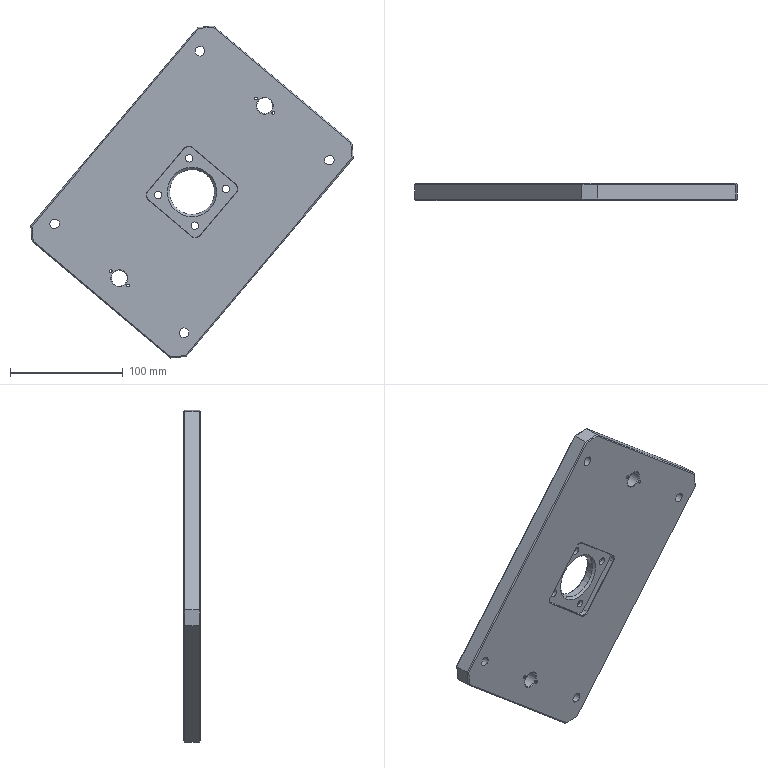Component | SolidWorks | 01GripperConnectionPlate-1 | 1 solid | 107 faces | box 285.83 x 15 x 294.29 mm | volume 624686 mm3 | cylinder 46 | plane 41 | cone 20 | commonest cylinder face diameters 2.5 x8 11 x8 6.6 x8 8.5 x8 14 x4 27 x4 10 x4 40 x2 | material Aviation Aluminum-7075
build123d program:
from build123d import *

# Parameters (mm, degrees)
SKETCH1_W                                          = 250
SKETCH1_H                                          = 180
BOSS_EXTRUDE1_DEPTH                                = 15
M10_TAPPED_HOLE1_D                                 = 8.5
SKETCH3_W                                          = 60
SKETCH3_H                                          = 60
CUT_EXTRUDE1_DEPTH                                 = 5
CHAMFER1_SIZE                                      = 10
FILLET1_R                                          = 5
CUT_EXTRUDE2_REACH                                 = 156.353
SKETCH4_R                                          = 20
CUT_EXTRUDE3_REACH                                 = 156.758
SKETCH5_R                                          = 5
HOLE_SIZE_ACCORDING_TO_TYPE_1_OF_HEXAG_D           = 6.6
HOLE_SIZE_ACCORDING_TO_TYPE_1_OF_HEXAG_CBORE_D     = 11
HOLE_SIZE_ACCORDING_TO_TYPE_1_OF_HEXAG_CBORE_DEPTH = 6.8
CIRPATTERN1_COUNT                                  = 4
CHAMFER2_SIZE                                      = 0.5
SKETCH7_R                                          = 13.5
CUT_EXTRUDE4_DEPTH                                 = 5
CUT_EXTRUDE5_REACH                                 = 156.353
SKETCH8_R                                          = 7
CHAMFER3_SIZE                                      = 0.5
M3_TAPPED_HOLE1_D                                  = 2.5
LPATTERN1_COUNT                                    = 2
LPATTERN1_PITCH                                    = 200
CHAMFER4_SIZE                                      = 1
CHAMFER5_SIZE                                      = 2


with BuildPart() as part:
    # Sketch1 → Boss-Extrude1 (new body)
    with BuildSketch(Plane.XY):
        Rectangle(SKETCH1_W, SKETCH1_H)
    extrude(amount=BOSS_EXTRUDE1_DEPTH)

    # M10 Tapped Hole1 (through all)
    with Locations(Plane(origin=(-100, 75, 15), x_dir=(1, 0, 0), z_dir=(0, 0, 1))):
        with Locations((0, 0), (0, -150), (200, -150), (200, 0)):
            Hole(M10_TAPPED_HOLE1_D / 2)

    # Sketch3 → Cut-Extrude1 (cut)
    with BuildSketch(Plane.XY.offset(15)):
        Rectangle(SKETCH3_W, SKETCH3_H)
    extrude(amount=-CUT_EXTRUDE1_DEPTH, mode=Mode.SUBTRACT)

    # Chamfer1
    chamfer1_edges = [part.edges().sort_by_distance(p)[0] for p in [
        (-125, 90, 7.5),
        (125, 90, 7.5),
        (125, -90, 7.5),
        (-125, -90, 7.5),
    ]]
    chamfer(chamfer1_edges, length=CHAMFER1_SIZE)

    # Fillet1
    fillet1_edges = [part.edges().sort_by_distance(p)[0] for p in [
        (-30, -30, 12.5),
        (-30, 30, 12.5),
        (30, 30, 12.5),
        (30, -30, 12.5),
    ]]
    fillet(fillet1_edges, radius=FILLET1_R)

    # Sketch4 → Cut-Extrude2 (cut, up to next)
    with BuildSketch(Plane.XY.offset(10), mode=Mode.PRIVATE) as cut_extrude2_sk1:
        Circle(SKETCH4_R)
    cut_extrude2_tool1 = extrude(cut_extrude2_sk1.sketch, amount=-CUT_EXTRUDE2_REACH, mode=Mode.PRIVATE) & part.part
    add(cut_extrude2_tool1.solids().sort_by_distance((0, 0, 10))[0], mode=Mode.SUBTRACT)

    # Sketch5 → Cut-Extrude3 (cut, up to next)
    with BuildSketch(Plane.XY.offset(15), mode=Mode.PRIVATE) as cut_extrude3_sk1:
        with Locations((-100, 0)):
            Circle(SKETCH5_R)
    cut_extrude3_tool1 = extrude(cut_extrude3_sk1.sketch, amount=-CUT_EXTRUDE3_REACH, mode=Mode.PRIVATE) & part.part
    # Sketch5 → Cut-Extrude3 (cut, up to next)
    with BuildSketch(Plane.XY.offset(15), mode=Mode.PRIVATE) as cut_extrude3_sk2:
        with Locations((100, 0)):
            Circle(SKETCH5_R)
    cut_extrude3_tool2 = extrude(cut_extrude3_sk2.sketch, amount=-CUT_EXTRUDE3_REACH, mode=Mode.PRIVATE) & part.part
    add(cut_extrude3_tool1.solids().sort_by_distance((-100, 0, 15))[0], mode=Mode.SUBTRACT)
    add(cut_extrude3_tool2.solids().sort_by_distance((100, 0, 15))[0], mode=Mode.SUBTRACT)

    # Hole Size _According to_ Type 1 of Hexag (through all)
    with Locations(Plane(origin=(21.213, 21.213, 0), x_dir=(-1, 0, 0), z_dir=(0, 0, -1))):
        with Locations((0, 0)):
            hole_size_according_to_type_1_of_hexag = CounterBoreHole(HOLE_SIZE_ACCORDING_TO_TYPE_1_OF_HEXAG_D / 2, HOLE_SIZE_ACCORDING_TO_TYPE_1_OF_HEXAG_CBORE_D / 2, HOLE_SIZE_ACCORDING_TO_TYPE_1_OF_HEXAG_CBORE_DEPTH)

    # CirPattern1: Hole Size _According to_ Type 1 of Hexag ×4 about axis
    cirpattern1_axis = Axis((0, 0, 0), (0, 0, 1))
    for i in range(1, CIRPATTERN1_COUNT):
        add(hole_size_according_to_type_1_of_hexag.rotate(cirpattern1_axis, i * 360 / CIRPATTERN1_COUNT), mode=Mode.SUBTRACT)

    # Chamfer2
    chamfer2_edges = [part.edges().sort_by_distance(p)[0] for p in [
        (30, 0, 15),
        (0, -30, 15),
        (-30, 0, 15),
        (0, 30, 15),
        (28.536, -28.536, 15),
        (-28.536, -28.536, 15),
        (-28.536, 28.536, 15),
        (28.536, 28.536, 15),
    ]]
    chamfer(chamfer2_edges, length=CHAMFER2_SIZE)

    # Sketch7 → Cut-Extrude4 (cut)
    with BuildSketch(Plane(origin=(0, 0, 0), x_dir=(-1, 0, 0), z_dir=(0, 0, -1))):
        with Locations((-100, 0)):
            Circle(SKETCH7_R)
        with Locations((100, 0)):
            Circle(SKETCH7_R)
    extrude(amount=-CUT_EXTRUDE4_DEPTH, mode=Mode.SUBTRACT)

    # Sketch8 → Cut-Extrude5 (cut, up to next)
    with BuildSketch(Plane(origin=(0, 0, 5), x_dir=(-1, 0, 0), z_dir=(0, 0, -1)), mode=Mode.PRIVATE) as cut_extrude5_sk1:
        with Locations((-100, 0)):
            Circle(SKETCH8_R)
    cut_extrude5_tool1 = extrude(cut_extrude5_sk1.sketch, amount=-CUT_EXTRUDE5_REACH, mode=Mode.PRIVATE) & part.part
    # Sketch8 → Cut-Extrude5 (cut, up to next)
    with BuildSketch(Plane(origin=(0, 0, 5), x_dir=(-1, 0, 0), z_dir=(0, 0, -1)), mode=Mode.PRIVATE) as cut_extrude5_sk2:
        with Locations((100, 0)):
            Circle(SKETCH8_R)
    cut_extrude5_tool2 = extrude(cut_extrude5_sk2.sketch, amount=-CUT_EXTRUDE5_REACH, mode=Mode.PRIVATE) & part.part
    add(cut_extrude5_tool1.solids().sort_by_distance((100, 0, 5))[0], mode=Mode.SUBTRACT)
    add(cut_extrude5_tool2.solids().sort_by_distance((-100, 0, 5))[0], mode=Mode.SUBTRACT)

    # Chamfer3
    chamfer3_edges = [part.edges().sort_by_distance(p)[0] for p in [
        (113.5, 0, 0),
        (-86.5, 0, 0),
        (107, 0, 15),
        (107, 0, 5),
        (-93, 0, 15),
        (-93, 0, 5),
    ]]
    chamfer(chamfer3_edges, length=CHAMFER3_SIZE)

    # M3 Tapped Hole1 (through all)
    with Locations(Plane(origin=(-100, 10, 5), x_dir=(-1, 0, 0), z_dir=(0, 0, -1))):
        with Locations((0, 0), (0, -20)):
            m3_tapped_hole1 = Hole(M3_TAPPED_HOLE1_D / 2)

    # LPattern1: M3 Tapped Hole1 ×2
    with Locations(*[(i * LPATTERN1_PITCH, 0, 0) for i in range(1, LPATTERN1_COUNT)]):
        add(m3_tapped_hole1, mode=Mode.SUBTRACT)

    # Chamfer4
    chamfer4_edges = [part.edges().sort_by_distance(p)[0] for p in [
        (0, -90, 0),
        (0, -90, 15),
        (-125, 0, 0),
        (0, 90, 0),
        (125, 0, 0),
        (-120, 85, 0),
        (120, 85, 0),
        (120, -85, 0),
        (-120, -85, 0),
        (-125, 0, 15),
        (125, 0, 15),
        (0, 90, 15),
        (-120, 85, 15),
        (120, 85, 15),
        (120, -85, 15),
        (-120, -85, 15),
    ]]
    chamfer(chamfer4_edges, length=CHAMFER4_SIZE)

    # Chamfer5
    chamfer5_edges = [part.edges().sort_by_distance(p)[0] for p in [
        (-20, 0, 10),
        (-20, 0, 0),
    ]]
    chamfer(chamfer5_edges, length=CHAMFER5_SIZE)


solid = part.part

# Placed as in the assembly
solid = solid.moved(Location((-144.488, 214.645, -264.11), (90, 0, 49.905)))